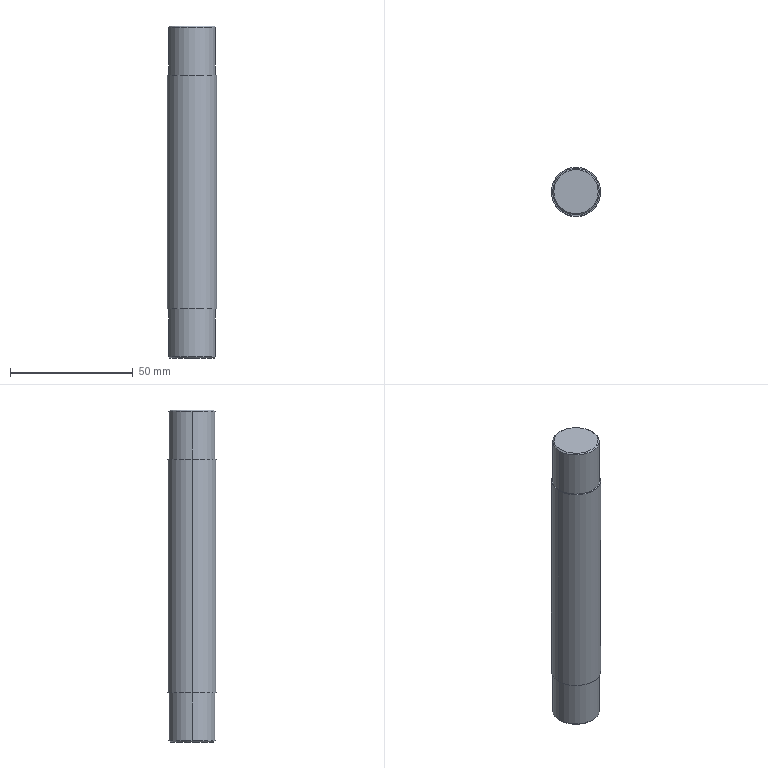Component | SolidWorks | TractionDrivenWheel-1_TractionDrivenWheelAxis-1 | 1 solid | 14 faces | box 20 x 20 x 135 mm | volume 41172 mm3 | cylinder 6 | cone 4 | plane 4 | commonest cylinder face diameters 19 x4 20 x2
build123d program:
from build123d import *

# Parameters (mm, degrees)
SKETCH1_R           = 10
BOSS_EXTRUDE1_DEPTH = 67.5
SKETCH2_R           = 10
SKETCH2_R_2         = 9.5
CUT_EXTRUDE1_DEPTH  = 20
CHAMFER1_SIZE       = 0.5


with BuildPart() as part:
    # Sketch1 → Boss-Extrude1 (new, symmetric)
    with BuildSketch(Plane(origin=(0, 0, 0), x_dir=(0, 0, -1), z_dir=(1, 0, 0))):
        Circle(SKETCH1_R)
    extrude(amount=BOSS_EXTRUDE1_DEPTH, both=True)

    # Sketch2 → Cut-Extrude1 (cut)
    with BuildSketch(Plane(origin=(67.5, 0, 0), x_dir=(0, 0, -1), z_dir=(1, 0, 0))):
        Circle(SKETCH2_R)
        Circle(SKETCH2_R_2, mode=Mode.SUBTRACT)
    cut_extrude1 = extrude(amount=-CUT_EXTRUDE1_DEPTH, mode=Mode.SUBTRACT)

    # Mirror1: Cut-Extrude1 across plane
    add(cut_extrude1.mirror(Plane(origin=(0, 0, 0), x_dir=(0, 0, 1), z_dir=(1, 0, 0))), mode=Mode.SUBTRACT)

    # Chamfer1
    chamfer1_edges = [part.edges().sort_by_distance(p)[0] for p in [
        (-67.5, 0, 9.5),
        (67.5, 0, 9.5),
    ]]
    chamfer(chamfer1_edges, length=CHAMFER1_SIZE)


solid = part.part

# Placed as in the assembly
solid = solid.moved(Location((225.493, -197.911, 568.5), (0, 90, 0)))
STEP:
#1=COLOUR_RGB('',0.7922,0.8196,0.9333);
#2=FILL_AREA_STYLE_COLOUR('',#1);
#3=FILL_AREA_STYLE('',(#2));
#4=SURFACE_STYLE_FILL_AREA(#3);
#5=SURFACE_SIDE_STYLE('',(#4));
#6=SURFACE_STYLE_USAGE(.BOTH.,#5);
#7=PRESENTATION_STYLE_ASSIGNMENT((#6));
#8=CARTESIAN_POINT('',(8.523,-7.792,19.724));
#9=VERTEX_POINT('',#8);
#10=CARTESIAN_POINT('',(9.232,-7.792,19.724));
#11=VERTEX_POINT('',#10);
#12=CARTESIAN_POINT('',(8.878,-7.792,19.724));
#13=DIRECTION('',(0.,0.,-1.));
#14=DIRECTION('',(1.,0.,0.));
#15=AXIS2_PLACEMENT_3D('',#12,#13,#14);
#16=CIRCLE('',#15,0.3543);
#17=EDGE_CURVE('',#9,#11,#16,.T.);
#18=ORIENTED_EDGE('',*,*,#17,.F.);
#19=CARTESIAN_POINT('',(8.504,-7.792,19.744));
#20=VERTEX_POINT('',#19);
#21=CARTESIAN_POINT('',(8.504,-7.792,19.744));
#22=DIRECTION('',(-0.7071,0.,0.7071));
#23=VECTOR('',#22,39.37);
#24=LINE('',#21,#23);
#25=EDGE_CURVE('',#9,#20,#24,.T.);
#26=ORIENTED_EDGE('',*,*,#25,.T.);
#27=CARTESIAN_POINT('',(9.252,-7.792,19.744));
#28=VERTEX_POINT('',#27);
#29=CARTESIAN_POINT('',(8.878,-7.792,19.744));
#30=DIRECTION('',(0.,0.,1.));
#31=DIRECTION('',(1.,0.,0.));
#32=AXIS2_PLACEMENT_3D('',#29,#30,#31);
#33=CIRCLE('',#32,0.374);
#34=EDGE_CURVE('',#28,#20,#33,.T.);
#35=ORIENTED_EDGE('',*,*,#34,.F.);
#36=CARTESIAN_POINT('',(9.252,-7.792,19.744));
#37=DIRECTION('',(0.7071,0.,0.7071));
#38=VECTOR('',#37,39.37);
#39=LINE('',#36,#38);
#40=EDGE_CURVE('',#11,#28,#39,.T.);
#41=ORIENTED_EDGE('',*,*,#40,.F.);
#42=EDGE_LOOP('',(#18,#26,#35,#41));
#43=FACE_OUTER_BOUND('',#42,.T.);
#44=CARTESIAN_POINT('',(8.878,-7.792,19.744));
#45=DIRECTION('',(0.,0.,1.));
#46=DIRECTION('',(1.,0.,0.));
#47=AXIS2_PLACEMENT_3D('',#44,#45,#46);
#48=CONICAL_SURFACE('',#47,0.374,0.7854);
#49=ADVANCED_FACE('',(#43),#48,.T.);
#50=CARTESIAN_POINT('',(9.232,-7.792,25.039));
#51=VERTEX_POINT('',#50);
#52=CARTESIAN_POINT('',(8.523,-7.792,25.039));
#53=VERTEX_POINT('',#52);
#54=CARTESIAN_POINT('',(8.878,-7.792,25.039));
#55=DIRECTION('',(0.,0.,1.));
#56=DIRECTION('',(1.,0.,0.));
#57=AXIS2_PLACEMENT_3D('',#54,#55,#56);
#58=CIRCLE('',#57,0.3543);
#59=EDGE_CURVE('',#51,#53,#58,.T.);
#60=ORIENTED_EDGE('',*,*,#59,.F.);
#61=CARTESIAN_POINT('',(9.252,-7.792,25.02));
#62=VERTEX_POINT('',#61);
#63=CARTESIAN_POINT('',(9.232,-7.792,25.039));
#64=DIRECTION('',(0.7071,0.,-0.7071));
#65=VECTOR('',#64,39.37);
#66=LINE('',#63,#65);
#67=EDGE_CURVE('',#51,#62,#66,.T.);
#68=ORIENTED_EDGE('',*,*,#67,.T.);
#69=CARTESIAN_POINT('',(8.504,-7.792,25.02));
#70=VERTEX_POINT('',#69);
#71=CARTESIAN_POINT('',(8.878,-7.792,25.02));
#72=DIRECTION('',(0.,0.,-1.));
#73=DIRECTION('',(1.,0.,0.));
#74=AXIS2_PLACEMENT_3D('',#71,#72,#73);
#75=CIRCLE('',#74,0.374);
#76=EDGE_CURVE('',#70,#62,#75,.T.);
#77=ORIENTED_EDGE('',*,*,#76,.F.);
#78=CARTESIAN_POINT('',(8.523,-7.792,25.039));
#79=DIRECTION('',(-0.7071,-0.,-0.7071));
#80=VECTOR('',#79,39.37);
#81=LINE('',#78,#80);
#82=EDGE_CURVE('',#53,#70,#81,.T.);
#83=ORIENTED_EDGE('',*,*,#82,.F.);
#84=EDGE_LOOP('',(#60,#68,#77,#83));
#85=FACE_OUTER_BOUND('',#84,.T.);
#86=CARTESIAN_POINT('',(8.878,-7.792,25.039));
#87=DIRECTION('',(0.,0.,-1.));
#88=DIRECTION('',(-1.,0.,0.));
#89=AXIS2_PLACEMENT_3D('',#86,#87,#88);
#90=CONICAL_SURFACE('',#89,0.3543,0.7854);
#91=ADVANCED_FACE('',(#85),#90,.T.);
#92=CARTESIAN_POINT('',(9.252,-7.792,20.512));
#93=VERTEX_POINT('',#92);
#94=CARTESIAN_POINT('',(8.504,-7.792,20.512));
#95=VERTEX_POINT('',#94);
#96=CARTESIAN_POINT('',(8.878,-7.792,20.512));
#97=DIRECTION('',(0.,0.,1.));
#98=DIRECTION('',(1.,0.,0.));
#99=AXIS2_PLACEMENT_3D('',#96,#97,#98);
#100=CIRCLE('',#99,0.374);
#101=EDGE_CURVE('',#93,#95,#100,.T.);
#102=ORIENTED_EDGE('',*,*,#101,.F.);
#103=CARTESIAN_POINT('',(9.252,-7.792,20.512));
#104=DIRECTION('',(0.,0.,-1.));
#105=VECTOR('',#104,39.37);
#106=LINE('',#103,#105);
#107=EDGE_CURVE('',#93,#28,#106,.T.);
#108=ORIENTED_EDGE('',*,*,#107,.T.);
#109=ORIENTED_EDGE('',*,*,#34,.T.);
#110=CARTESIAN_POINT('',(8.504,-7.792,20.512));
#111=DIRECTION('',(0.,0.,-1.));
#112=VECTOR('',#111,39.37);
#113=LINE('',#110,#112);
#114=EDGE_CURVE('',#95,#20,#113,.T.);
#115=ORIENTED_EDGE('',*,*,#114,.F.);
#116=EDGE_LOOP('',(#102,#108,#109,#115));
#117=FACE_OUTER_BOUND('',#116,.T.);
#118=CARTESIAN_POINT('',(8.878,-7.792,20.512));
#119=DIRECTION('',(0.,0.,-1.));
#120=DIRECTION('',(-1.,0.,0.));
#121=AXIS2_PLACEMENT_3D('',#118,#119,#120);
#122=CYLINDRICAL_SURFACE('',#121,0.374);
#123=ADVANCED_FACE('',(#117),#122,.T.);
#124=CARTESIAN_POINT('',(9.252,-7.792,24.252));
#125=VERTEX_POINT('',#124);
#126=CARTESIAN_POINT('',(8.504,-7.792,24.252));
#127=VERTEX_POINT('',#126);
#128=CARTESIAN_POINT('',(8.878,-7.792,24.252));
#129=DIRECTION('',(0.,0.,1.));
#130=DIRECTION('',(1.,0.,0.));
#131=AXIS2_PLACEMENT_3D('',#128,#129,#130);
#132=CIRCLE('',#131,0.374);
#133=EDGE_CURVE('',#125,#127,#132,.T.);
#134=ORIENTED_EDGE('',*,*,#133,.T.);
#135=CARTESIAN_POINT('',(8.504,-7.792,24.252));
#136=DIRECTION('',(0.,0.,1.));
#137=VECTOR('',#136,39.37);
#138=LINE('',#135,#137);
#139=EDGE_CURVE('',#127,#70,#138,.T.);
#140=ORIENTED_EDGE('',*,*,#139,.T.);
#141=ORIENTED_EDGE('',*,*,#76,.T.);
#142=CARTESIAN_POINT('',(9.252,-7.792,24.252));
#143=DIRECTION('',(0.,0.,1.));
#144=VECTOR('',#143,39.37);
#145=LINE('',#142,#144);
#146=EDGE_CURVE('',#125,#62,#145,.T.);
#147=ORIENTED_EDGE('',*,*,#146,.F.);
#148=EDGE_LOOP('',(#134,#140,#141,#147));
#149=FACE_OUTER_BOUND('',#148,.T.);
#150=CARTESIAN_POINT('',(8.878,-7.792,24.252));
#151=DIRECTION('',(0.,0.,1.));
#152=DIRECTION('',(1.,0.,0.));
#153=AXIS2_PLACEMENT_3D('',#150,#151,#152);
#154=CYLINDRICAL_SURFACE('',#153,0.374);
#155=ADVANCED_FACE('',(#149),#154,.T.);
#156=CARTESIAN_POINT('',(9.271,-7.792,24.252));
#157=VERTEX_POINT('',#156);
#158=CARTESIAN_POINT('',(8.484,-7.792,24.252));
#159=VERTEX_POINT('',#158);
#160=CARTESIAN_POINT('',(8.878,-7.792,24.252));
#161=DIRECTION('',(0.,0.,1.));
#162=DIRECTION('',(1.,0.,0.));
#163=AXIS2_PLACEMENT_3D('',#160,#161,#162);
#164=CIRCLE('',#163,0.3937);
#165=EDGE_CURVE('',#157,#159,#164,.T.);
#166=ORIENTED_EDGE('',*,*,#165,.F.);
#167=CARTESIAN_POINT('',(9.271,-7.792,20.512));
#168=VERTEX_POINT('',#167);
#169=CARTESIAN_POINT('',(9.271,-7.792,25.039));
#170=DIRECTION('',(0.,0.,-1.));
#171=VECTOR('',#170,39.37);
#172=LINE('',#169,#171);
#173=EDGE_CURVE('',#157,#168,#172,.T.);
#174=ORIENTED_EDGE('',*,*,#173,.T.);
#175=CARTESIAN_POINT('',(8.484,-7.792,20.512));
#176=VERTEX_POINT('',#175);
#177=CARTESIAN_POINT('',(8.878,-7.792,20.512));
#178=DIRECTION('',(0.,0.,1.));
#179=DIRECTION('',(1.,0.,0.));
#180=AXIS2_PLACEMENT_3D('',#177,#178,#179);
#181=CIRCLE('',#180,0.3937);
#182=EDGE_CURVE('',#168,#176,#181,.T.);
#183=ORIENTED_EDGE('',*,*,#182,.T.);
#184=CARTESIAN_POINT('',(8.484,-7.792,25.039));
#185=DIRECTION('',(0.,0.,-1.));
#186=VECTOR('',#185,39.37);
#187=LINE('',#184,#186);
#188=EDGE_CURVE('',#159,#176,#187,.T.);
#189=ORIENTED_EDGE('',*,*,#188,.F.);
#190=EDGE_LOOP('',(#166,#174,#183,#189));
#191=FACE_OUTER_BOUND('',#190,.T.);
#192=CARTESIAN_POINT('',(8.878,-7.792,25.039));
#193=DIRECTION('',(0.,0.,-1.));
#194=DIRECTION('',(-1.,0.,0.));
#195=AXIS2_PLACEMENT_3D('',#192,#193,#194);
#196=CYLINDRICAL_SURFACE('',#195,0.3937);
#197=ADVANCED_FACE('',(#191),#196,.T.);
#198=ORIENTED_EDGE('',*,*,#173,.F.);
#199=CARTESIAN_POINT('',(8.878,-7.792,24.252));
#200=DIRECTION('',(0.,0.,1.));
#201=DIRECTION('',(1.,0.,0.));
#202=AXIS2_PLACEMENT_3D('',#199,#200,#201);
#203=CIRCLE('',#202,0.3937);
#204=EDGE_CURVE('',#159,#157,#203,.T.);
#205=ORIENTED_EDGE('',*,*,#204,.F.);
#206=ORIENTED_EDGE('',*,*,#188,.T.);
#207=CARTESIAN_POINT('',(8.878,-7.792,20.512));
#208=DIRECTION('',(0.,0.,1.));
#209=DIRECTION('',(1.,0.,0.));
#210=AXIS2_PLACEMENT_3D('',#207,#208,#209);
#211=CIRCLE('',#210,0.3937);
#212=EDGE_CURVE('',#176,#168,#211,.T.);
#213=ORIENTED_EDGE('',*,*,#212,.T.);
#214=EDGE_LOOP('',(#198,#205,#206,#213));
#215=FACE_OUTER_BOUND('',#214,.T.);
#216=CARTESIAN_POINT('',(8.878,-7.792,25.039));
#217=DIRECTION('',(0.,0.,-1.));
#218=DIRECTION('',(-1.,0.,0.));
#219=AXIS2_PLACEMENT_3D('',#216,#217,#218);
#220=CYLINDRICAL_SURFACE('',#219,0.3937);
#221=ADVANCED_FACE('',(#215),#220,.T.);
#222=ORIENTED_EDGE('',*,*,#133,.F.);
#223=CARTESIAN_POINT('',(8.878,-7.792,24.252));
#224=DIRECTION('',(0.,0.,1.));
#225=DIRECTION('',(1.,0.,0.));
#226=AXIS2_PLACEMENT_3D('',#223,#224,#225);
#227=CIRCLE('',#226,0.374);
#228=EDGE_CURVE('',#127,#125,#227,.T.);
#229=ORIENTED_EDGE('',*,*,#228,.F.);
#230=EDGE_LOOP('',(#222,#229));
#231=FACE_BOUND('',#230,.T.);
#232=ORIENTED_EDGE('',*,*,#204,.T.);
#233=ORIENTED_EDGE('',*,*,#165,.T.);
#234=EDGE_LOOP('',(#232,#233));
#235=FACE_OUTER_BOUND('',#234,.T.);
#236=CARTESIAN_POINT('',(8.878,-7.792,24.252));
#237=DIRECTION('',(0.,0.,1.));
#238=DIRECTION('',(1.,0.,0.));
#239=AXIS2_PLACEMENT_3D('',#236,#237,#238);
#240=PLANE('',#239);
#241=ADVANCED_FACE('',(#231,#235),#240,.T.);
#242=ORIENTED_EDGE('',*,*,#139,.F.);
#243=ORIENTED_EDGE('',*,*,#228,.T.);
#244=ORIENTED_EDGE('',*,*,#146,.T.);
#245=CARTESIAN_POINT('',(8.878,-7.792,25.02));
#246=DIRECTION('',(0.,0.,-1.));
#247=DIRECTION('',(1.,0.,0.));
#248=AXIS2_PLACEMENT_3D('',#245,#246,#247);
#249=CIRCLE('',#248,0.374);
#250=EDGE_CURVE('',#62,#70,#249,.T.);
#251=ORIENTED_EDGE('',*,*,#250,.T.);
#252=EDGE_LOOP('',(#242,#243,#244,#251));
#253=FACE_OUTER_BOUND('',#252,.T.);
#254=CARTESIAN_POINT('',(8.878,-7.792,24.252));
#255=DIRECTION('',(0.,0.,1.));
#256=DIRECTION('',(1.,0.,0.));
#257=AXIS2_PLACEMENT_3D('',#254,#255,#256);
#258=CYLINDRICAL_SURFACE('',#257,0.374);
#259=ADVANCED_FACE('',(#253),#258,.T.);
#260=CARTESIAN_POINT('',(8.878,-7.792,25.039));
#261=DIRECTION('',(0.,0.,1.));
#262=DIRECTION('',(1.,0.,0.));
#263=AXIS2_PLACEMENT_3D('',#260,#261,#262);
#264=CIRCLE('',#263,0.3543);
#265=EDGE_CURVE('',#53,#51,#264,.T.);
#266=ORIENTED_EDGE('',*,*,#265,.T.);
#267=ORIENTED_EDGE('',*,*,#59,.T.);
#268=EDGE_LOOP('',(#266,#267));
#269=FACE_OUTER_BOUND('',#268,.T.);
#270=CARTESIAN_POINT('',(8.878,-7.792,25.039));
#271=DIRECTION('',(0.,0.,1.));
#272=DIRECTION('',(1.,0.,0.));
#273=AXIS2_PLACEMENT_3D('',#270,#271,#272);
#274=PLANE('',#273);
#275=ADVANCED_FACE('',(#269),#274,.T.);
#276=ORIENTED_EDGE('',*,*,#212,.F.);
#277=ORIENTED_EDGE('',*,*,#182,.F.);
#278=EDGE_LOOP('',(#276,#277));
#279=FACE_OUTER_BOUND('',#278,.T.);
#280=CARTESIAN_POINT('',(8.878,-7.792,20.512));
#281=DIRECTION('',(0.,0.,1.));
#282=DIRECTION('',(1.,0.,0.));
#283=AXIS2_PLACEMENT_3D('',#280,#281,#282);
#284=CIRCLE('',#283,0.374);
#285=EDGE_CURVE('',#95,#93,#284,.T.);
#286=ORIENTED_EDGE('',*,*,#285,.T.);
#287=ORIENTED_EDGE('',*,*,#101,.T.);
#288=EDGE_LOOP('',(#286,#287));
#289=FACE_BOUND('',#288,.T.);
#290=CARTESIAN_POINT('',(8.878,-7.792,20.512));
#291=DIRECTION('',(0.,0.,-1.));
#292=DIRECTION('',(1.,0.,0.));
#293=AXIS2_PLACEMENT_3D('',#290,#291,#292);
#294=PLANE('',#293);
#295=ADVANCED_FACE('',(#279,#289),#294,.T.);
#296=ORIENTED_EDGE('',*,*,#107,.F.);
#297=ORIENTED_EDGE('',*,*,#285,.F.);
#298=ORIENTED_EDGE('',*,*,#114,.T.);
#299=CARTESIAN_POINT('',(8.878,-7.792,19.744));
#300=DIRECTION('',(0.,0.,1.));
#301=DIRECTION('',(1.,0.,0.));
#302=AXIS2_PLACEMENT_3D('',#299,#300,#301);
#303=CIRCLE('',#302,0.374);
#304=EDGE_CURVE('',#20,#28,#303,.T.);
#305=ORIENTED_EDGE('',*,*,#304,.T.);
#306=EDGE_LOOP('',(#296,#297,#298,#305));
#307=FACE_OUTER_BOUND('',#306,.T.);
#308=CARTESIAN_POINT('',(8.878,-7.792,20.512));
#309=DIRECTION('',(0.,0.,-1.));
#310=DIRECTION('',(-1.,0.,0.));
#311=AXIS2_PLACEMENT_3D('',#308,#309,#310);
#312=CYLINDRICAL_SURFACE('',#311,0.374);
#313=ADVANCED_FACE('',(#307),#312,.T.);
#314=CARTESIAN_POINT('',(8.878,-7.792,19.724));
#315=DIRECTION('',(0.,0.,-1.));
#316=DIRECTION('',(1.,0.,0.));
#317=AXIS2_PLACEMENT_3D('',#314,#315,#316);
#318=CIRCLE('',#317,0.3543);
#319=EDGE_CURVE('',#11,#9,#318,.T.);
#320=ORIENTED_EDGE('',*,*,#319,.T.);
#321=ORIENTED_EDGE('',*,*,#17,.T.);
#322=EDGE_LOOP('',(#320,#321));
#323=FACE_OUTER_BOUND('',#322,.T.);
#324=CARTESIAN_POINT('',(8.878,-7.792,19.724));
#325=DIRECTION('',(0.,0.,1.));
#326=DIRECTION('',(1.,0.,0.));
#327=AXIS2_PLACEMENT_3D('',#324,#325,#326);
#328=PLANE('',#327);
#329=ADVANCED_FACE('',(#323),#328,.F.);
#330=ORIENTED_EDGE('',*,*,#67,.F.);
#331=ORIENTED_EDGE('',*,*,#265,.F.);
#332=ORIENTED_EDGE('',*,*,#82,.T.);
#333=ORIENTED_EDGE('',*,*,#250,.F.);
#334=EDGE_LOOP('',(#330,#331,#332,#333));
#335=FACE_OUTER_BOUND('',#334,.T.);
#336=CARTESIAN_POINT('',(8.878,-7.792,25.039));
#337=DIRECTION('',(0.,0.,-1.));
#338=DIRECTION('',(-1.,0.,0.));
#339=AXIS2_PLACEMENT_3D('',#336,#337,#338);
#340=CONICAL_SURFACE('',#339,0.3543,0.7854);
#341=ADVANCED_FACE('',(#335),#340,.T.);
#342=ORIENTED_EDGE('',*,*,#25,.F.);
#343=ORIENTED_EDGE('',*,*,#319,.F.);
#344=ORIENTED_EDGE('',*,*,#40,.T.);
#345=ORIENTED_EDGE('',*,*,#304,.F.);
#346=EDGE_LOOP('',(#342,#343,#344,#345));
#347=FACE_OUTER_BOUND('',#346,.T.);
#348=CARTESIAN_POINT('',(8.878,-7.792,19.744));
#349=DIRECTION('',(0.,0.,1.));
#350=DIRECTION('',(1.,0.,0.));
#351=AXIS2_PLACEMENT_3D('',#348,#349,#350);
#352=CONICAL_SURFACE('',#351,0.374,0.7854);
#353=ADVANCED_FACE('',(#347),#352,.T.);
#354=CLOSED_SHELL('',(#49,#91,#123,#155,#197,#221,#241,#259,#275,#295,#313,#329,#341,#353));
#355=MANIFOLD_SOLID_BREP('',#354);
#356=STYLED_ITEM('',(#7),#355);
#357=PRESENTATION_LAYER_ASSIGNMENT('','',(#356));
#358=(LENGTH_UNIT()NAMED_UNIT(*)SI_UNIT($,.METRE.));
#359=LENGTH_MEASURE_WITH_UNIT(LENGTH_MEASURE(0.0254),#358);
#360=DIMENSIONAL_EXPONENTS(1.,0.,0.,0.,0.,0.,0.);
#361=(CONVERSION_BASED_UNIT('',#359)LENGTH_UNIT()NAMED_UNIT(#360));
#362=UNCERTAINTY_MEASURE_WITH_UNIT(LENGTH_MEASURE(0.00001),#361,'','');
#363=(NAMED_UNIT(*)PLANE_ANGLE_UNIT()SI_UNIT($,.RADIAN.));
#364=(NAMED_UNIT(*)SI_UNIT($,.STERADIAN.)SOLID_ANGLE_UNIT());
#365=(GEOMETRIC_REPRESENTATION_CONTEXT(3)GLOBAL_UNCERTAINTY_ASSIGNED_CONTEXT((#362))GLOBAL_UNIT_ASSIGNED_CONTEXT((#361,#363,#364))REPRESENTATION_CONTEXT('',''));
#366=MECHANICAL_DESIGN_GEOMETRIC_PRESENTATION_REPRESENTATION('',(#356),#365);
#367=CARTESIAN_POINT('',(0.,0.,0.));
#368=DIRECTION('',(0.,0.,1.));
#369=DIRECTION('',(1.,0.,0.));
#370=AXIS2_PLACEMENT_3D('',#367,#368,#369);
#371=(LENGTH_UNIT()NAMED_UNIT(*)SI_UNIT($,.METRE.));
#372=LENGTH_MEASURE_WITH_UNIT(LENGTH_MEASURE(0.0254),#371);
#373=DIMENSIONAL_EXPONENTS(1.,0.,0.,0.,0.,0.,0.);
#374=(CONVERSION_BASED_UNIT('',#372)LENGTH_UNIT()NAMED_UNIT(#373));
#375=UNCERTAINTY_MEASURE_WITH_UNIT(LENGTH_MEASURE(0.00001),#374,'','');
#376=(NAMED_UNIT(*)PLANE_ANGLE_UNIT()SI_UNIT($,.RADIAN.));
#377=(NAMED_UNIT(*)SI_UNIT($,.STERADIAN.)SOLID_ANGLE_UNIT());
#378=(GEOMETRIC_REPRESENTATION_CONTEXT(3)GLOBAL_UNCERTAINTY_ASSIGNED_CONTEXT((#375))GLOBAL_UNIT_ASSIGNED_CONTEXT((#374,#376,#377))REPRESENTATION_CONTEXT('',''));
#379=ADVANCED_BREP_SHAPE_REPRESENTATION('',(#355,#370),#378);